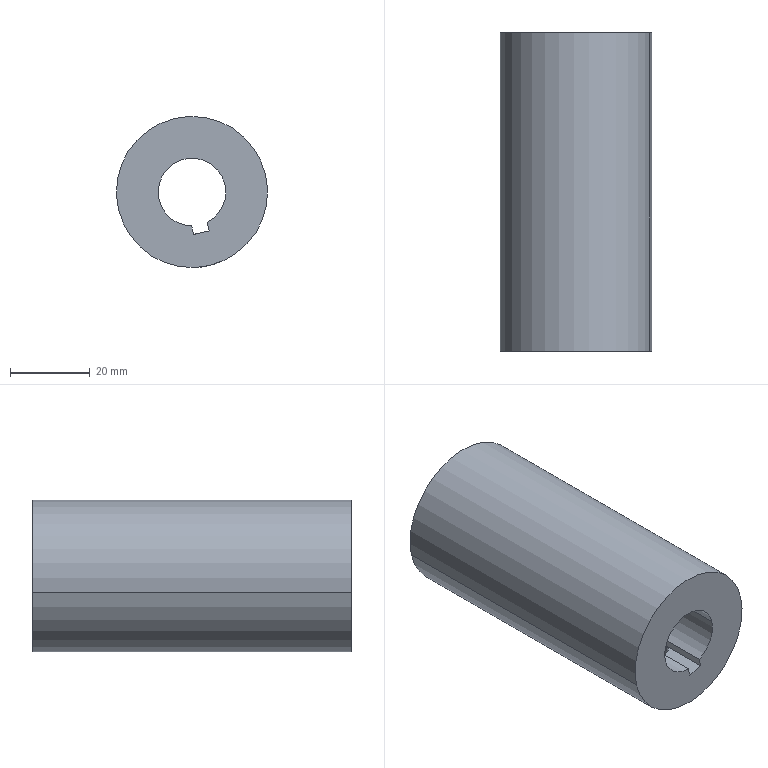Component | SolidWorks | Coupling1-1 | 1 solid | 20 faces | box 38 x 80 x 38 mm | volume 71671 mm3 | plane 11 | cylinder 9 | commonest cylinder face diameters 4.2 x4 17 x3 38 x2
build123d program:
from build123d import *

# Parameters (mm, degrees)
SKETCH1_R                  = 19
EXTRUDE1_DEPTH             = 80
M5_TAPPED_HOLE1_AT_2_COUNT = 2
M5_TAPPED_HOLE1_AT_2_PITCH = 55


with BuildPart() as part:
    # Sketch1 → Extrude1 (new body)
    with BuildSketch(Plane(origin=(0, 0, 0), x_dir=(1, 0, 0), z_dir=(0, 1, 0))):
        with Locations(Location((0, 0, 0), (0, 0, 270))):
            Circle(SKETCH1_R)
        with BuildLine():
            Line((8.261, 2), (10.5, 2))
            Line((10.5, 2), (10.5, -2))
            Line((10.5, -2), (8.261, -2))
            ThreePointArc((8.261, -2), (-8.5, 0), (8.261, 2))
        make_face(mode=Mode.SUBTRACT)
    extrude(amount=EXTRUDE1_DEPTH)

    # Sketch2 → M5 Tapped Hole1 (revolve, cut)
    with BuildSketch(Plane(origin=(10.5, 67.5, 0), x_dir=(0, 0, 1), z_dir=(0, 1, 0))):
        Polygon((0, 0), (0, 15.262), (2.1, 14), (2.1, 0), align=None)
    m5_tapped_hole1 = revolve(axis=Axis((4.15, 67.5, 0), (1, 0, 0)), mode=Mode.SUBTRACT)

    # M5 Tapped Hole1 at 2: M5 Tapped Hole1 ×2
    with Locations(*[(0, -i * M5_TAPPED_HOLE1_AT_2_PITCH, 0) for i in range(1, M5_TAPPED_HOLE1_AT_2_COUNT)]):
        add(m5_tapped_hole1, mode=Mode.SUBTRACT)


solid = part.part

# Placed as in the assembly
solid = solid.moved(Location((-164.784, 235.983, 4), (0, 77.072, 0)))
STEP:
#1=CARTESIAN_POINT('',(-6.402,11.948,-0.5856));
#2=VERTEX_POINT('',#1);
#3=CARTESIAN_POINT('',(-6.241,11.948,-0.5486));
#4=VERTEX_POINT('',#3);
#5=CARTESIAN_POINT('',(-6.402,11.948,-0.5856));
#6=CARTESIAN_POINT('',(-6.402,11.937,-0.5856));
#7=CARTESIAN_POINT('',(-6.4,11.926,-0.5854));
#8=CARTESIAN_POINT('',(-6.391,11.907,-0.5843));
#9=CARTESIAN_POINT('',(-6.385,11.897,-0.5836));
#10=CARTESIAN_POINT('',(-6.374,11.886,-0.5819));
#11=CARTESIAN_POINT('',(-6.37,11.882,-0.5812));
#12=CARTESIAN_POINT('',(-6.361,11.876,-0.5797));
#13=CARTESIAN_POINT('',(-6.356,11.874,-0.5789));
#14=CARTESIAN_POINT('',(-6.346,11.87,-0.5771));
#15=CARTESIAN_POINT('',(-6.341,11.868,-0.5761));
#16=CARTESIAN_POINT('',(-6.331,11.866,-0.574));
#17=CARTESIAN_POINT('',(-6.325,11.865,-0.5728));
#18=CARTESIAN_POINT('',(-6.315,11.865,-0.5704));
#19=CARTESIAN_POINT('',(-6.31,11.866,-0.5691));
#20=CARTESIAN_POINT('',(-6.299,11.868,-0.5665));
#21=CARTESIAN_POINT('',(-6.294,11.87,-0.5652));
#22=CARTESIAN_POINT('',(-6.285,11.874,-0.5625));
#23=CARTESIAN_POINT('',(-6.28,11.876,-0.5612));
#24=CARTESIAN_POINT('',(-6.271,11.882,-0.5587));
#25=CARTESIAN_POINT('',(-6.267,11.886,-0.5574));
#26=CARTESIAN_POINT('',(-6.256,11.897,-0.554));
#27=CARTESIAN_POINT('',(-6.251,11.906,-0.552));
#28=CARTESIAN_POINT('',(-6.243,11.926,-0.5493));
#29=CARTESIAN_POINT('',(-6.241,11.937,-0.5486));
#30=CARTESIAN_POINT('',(-6.241,11.948,-0.5486));
#31=B_SPLINE_CURVE_WITH_KNOTS('',3,(#5,#6,#7,#8,#9,#10,#11,#12,#13,#14,#15,#16,#17,#18,#19,#20,#21,#22,#23,#24,#25,#26,#27,#28,#29,#30),.UNSPECIFIED.,.F.,.F.,(4,2,2,2,2,2,2,2,2,2,2,2,4),(0.006571,0.007392,0.008213,0.008623,0.009034,0.009445,0.009855,0.01027,0.01068,0.01109,0.0115,0.01232,0.01314),.UNSPECIFIED.);
#32=EDGE_CURVE('',#2,#4,#31,.T.);
#33=ORIENTED_EDGE('',*,*,#32,.F.);
#34=CARTESIAN_POINT('',(-6.476,11.948,-0.2639));
#35=VERTEX_POINT('',#34);
#36=CARTESIAN_POINT('',(-6.476,11.948,-0.2639));
#37=DIRECTION('',(-0.2238,0.,0.9746));
#38=VECTOR('',#37,39.37);
#39=LINE('',#36,#38);
#40=EDGE_CURVE('',#2,#35,#39,.T.);
#41=ORIENTED_EDGE('',*,*,#40,.T.);
#42=CARTESIAN_POINT('',(-6.472,11.923,-0.263));
#43=VERTEX_POINT('',#42);
#44=CARTESIAN_POINT('',(-6.395,11.948,-0.2454));
#45=DIRECTION('',(-0.2238,0.,0.9746));
#46=DIRECTION('',(0.9746,0.,0.2238));
#47=AXIS2_PLACEMENT_3D('',#44,#45,#46);
#48=CIRCLE('',#47,0.08268);
#49=EDGE_CURVE('',#35,#43,#48,.T.);
#50=ORIENTED_EDGE('',*,*,#49,.T.);
#51=CARTESIAN_POINT('',(-6.318,11.923,-0.2278));
#52=VERTEX_POINT('',#51);
#53=CARTESIAN_POINT('',(-6.395,11.948,-0.2454));
#54=DIRECTION('',(-0.2238,0.,0.9746));
#55=DIRECTION('',(0.9746,0.,0.2238));
#56=AXIS2_PLACEMENT_3D('',#53,#54,#55);
#57=CIRCLE('',#56,0.08268);
#58=EDGE_CURVE('',#43,#52,#57,.T.);
#59=ORIENTED_EDGE('',*,*,#58,.T.);
#60=CARTESIAN_POINT('',(-6.314,11.948,-0.2269));
#61=VERTEX_POINT('',#60);
#62=CARTESIAN_POINT('',(-6.395,11.948,-0.2454));
#63=DIRECTION('',(-0.2238,0.,0.9746));
#64=DIRECTION('',(0.9746,0.,0.2238));
#65=AXIS2_PLACEMENT_3D('',#62,#63,#64);
#66=CIRCLE('',#65,0.08268);
#67=EDGE_CURVE('',#52,#61,#66,.T.);
#68=ORIENTED_EDGE('',*,*,#67,.T.);
#69=CARTESIAN_POINT('',(-6.314,11.948,-0.2269));
#70=DIRECTION('',(-0.2238,0.,0.9746));
#71=VECTOR('',#70,39.37);
#72=LINE('',#69,#71);
#73=EDGE_CURVE('',#4,#61,#72,.T.);
#74=ORIENTED_EDGE('',*,*,#73,.F.);
#75=EDGE_LOOP('',(#33,#41,#50,#59,#68,#74));
#76=FACE_OUTER_BOUND('',#75,.T.);
#77=CARTESIAN_POINT('',(-6.395,11.948,-0.2454));
#78=DIRECTION('',(-0.2238,0.,0.9746));
#79=DIRECTION('',(0.9746,0.,0.2238));
#80=AXIS2_PLACEMENT_3D('',#77,#78,#79);
#81=CYLINDRICAL_SURFACE('',#80,0.08268);
#82=ADVANCED_FACE('',(#76),#81,.F.);
#83=CARTESIAN_POINT('',(-6.402,9.783,-0.5856));
#84=VERTEX_POINT('',#83);
#85=CARTESIAN_POINT('',(-6.241,9.783,-0.5486));
#86=VERTEX_POINT('',#85);
#87=CARTESIAN_POINT('',(-6.402,9.783,-0.5856));
#88=CARTESIAN_POINT('',(-6.402,9.772,-0.5856));
#89=CARTESIAN_POINT('',(-6.4,9.761,-0.5854));
#90=CARTESIAN_POINT('',(-6.391,9.741,-0.5843));
#91=CARTESIAN_POINT('',(-6.385,9.732,-0.5836));
#92=CARTESIAN_POINT('',(-6.374,9.721,-0.5819));
#93=CARTESIAN_POINT('',(-6.37,9.717,-0.5812));
#94=CARTESIAN_POINT('',(-6.361,9.711,-0.5797));
#95=CARTESIAN_POINT('',(-6.356,9.709,-0.5789));
#96=CARTESIAN_POINT('',(-6.346,9.704,-0.5771));
#97=CARTESIAN_POINT('',(-6.341,9.703,-0.5761));
#98=CARTESIAN_POINT('',(-6.331,9.701,-0.574));
#99=CARTESIAN_POINT('',(-6.325,9.7,-0.5728));
#100=CARTESIAN_POINT('',(-6.315,9.7,-0.5704));
#101=CARTESIAN_POINT('',(-6.31,9.701,-0.5691));
#102=CARTESIAN_POINT('',(-6.299,9.703,-0.5665));
#103=CARTESIAN_POINT('',(-6.294,9.704,-0.5652));
#104=CARTESIAN_POINT('',(-6.285,9.708,-0.5625));
#105=CARTESIAN_POINT('',(-6.28,9.711,-0.5612));
#106=CARTESIAN_POINT('',(-6.271,9.717,-0.5587));
#107=CARTESIAN_POINT('',(-6.267,9.721,-0.5574));
#108=CARTESIAN_POINT('',(-6.256,9.732,-0.554));
#109=CARTESIAN_POINT('',(-6.251,9.741,-0.552));
#110=CARTESIAN_POINT('',(-6.243,9.761,-0.5493));
#111=CARTESIAN_POINT('',(-6.241,9.772,-0.5486));
#112=CARTESIAN_POINT('',(-6.241,9.783,-0.5486));
#113=B_SPLINE_CURVE_WITH_KNOTS('',3,(#87,#88,#89,#90,#91,#92,#93,#94,#95,#96,#97,#98,#99,#100,#101,#102,#103,#104,#105,#106,#107,#108,#109,#110,#111,#112),.UNSPECIFIED.,.F.,.F.,(4,2,2,2,2,2,2,2,2,2,2,2,4),(0.006571,0.007392,0.008213,0.008623,0.009034,0.009445,0.009855,0.01027,0.01068,0.01109,0.0115,0.01232,0.01314),.UNSPECIFIED.);
#114=EDGE_CURVE('',#84,#86,#113,.T.);
#115=ORIENTED_EDGE('',*,*,#114,.F.);
#116=CARTESIAN_POINT('',(-6.476,9.783,-0.2639));
#117=VERTEX_POINT('',#116);
#118=CARTESIAN_POINT('',(-6.476,9.783,-0.2639));
#119=DIRECTION('',(-0.2238,0.,0.9746));
#120=VECTOR('',#119,39.37);
#121=LINE('',#118,#120);
#122=EDGE_CURVE('',#84,#117,#121,.T.);
#123=ORIENTED_EDGE('',*,*,#122,.T.);
#124=CARTESIAN_POINT('',(-6.472,9.758,-0.263));
#125=VERTEX_POINT('',#124);
#126=CARTESIAN_POINT('',(-6.395,9.783,-0.2454));
#127=DIRECTION('',(-0.2238,0.,0.9746));
#128=DIRECTION('',(0.9746,0.,0.2238));
#129=AXIS2_PLACEMENT_3D('',#126,#127,#128);
#130=CIRCLE('',#129,0.08268);
#131=EDGE_CURVE('',#117,#125,#130,.T.);
#132=ORIENTED_EDGE('',*,*,#131,.T.);
#133=CARTESIAN_POINT('',(-6.318,9.758,-0.2278));
#134=VERTEX_POINT('',#133);
#135=CARTESIAN_POINT('',(-6.395,9.783,-0.2454));
#136=DIRECTION('',(-0.2238,0.,0.9746));
#137=DIRECTION('',(0.9746,0.,0.2238));
#138=AXIS2_PLACEMENT_3D('',#135,#136,#137);
#139=CIRCLE('',#138,0.08268);
#140=EDGE_CURVE('',#125,#134,#139,.T.);
#141=ORIENTED_EDGE('',*,*,#140,.T.);
#142=CARTESIAN_POINT('',(-6.314,9.783,-0.2269));
#143=VERTEX_POINT('',#142);
#144=CARTESIAN_POINT('',(-6.395,9.783,-0.2454));
#145=DIRECTION('',(-0.2238,0.,0.9746));
#146=DIRECTION('',(0.9746,0.,0.2238));
#147=AXIS2_PLACEMENT_3D('',#144,#145,#146);
#148=CIRCLE('',#147,0.08268);
#149=EDGE_CURVE('',#134,#143,#148,.T.);
#150=ORIENTED_EDGE('',*,*,#149,.T.);
#151=CARTESIAN_POINT('',(-6.314,9.783,-0.2269));
#152=DIRECTION('',(-0.2238,0.,0.9746));
#153=VECTOR('',#152,39.37);
#154=LINE('',#151,#153);
#155=EDGE_CURVE('',#86,#143,#154,.T.);
#156=ORIENTED_EDGE('',*,*,#155,.F.);
#157=EDGE_LOOP('',(#115,#123,#132,#141,#150,#156));
#158=FACE_OUTER_BOUND('',#157,.T.);
#159=CARTESIAN_POINT('',(-6.395,9.783,-0.2454));
#160=DIRECTION('',(-0.2238,0.,0.9746));
#161=DIRECTION('',(0.9746,0.,0.2238));
#162=AXIS2_PLACEMENT_3D('',#159,#160,#161);
#163=CYLINDRICAL_SURFACE('',#162,0.08268);
#164=ADVANCED_FACE('',(#158),#163,.F.);
#165=CARTESIAN_POINT('',(-6.814,12.44,0.08257));
#166=VERTEX_POINT('',#165);
#167=CARTESIAN_POINT('',(-6.161,12.44,0.2324));
#168=VERTEX_POINT('',#167);
#169=CARTESIAN_POINT('',(-6.488,12.44,0.1575));
#170=DIRECTION('',(0.,1.,0.));
#171=DIRECTION('',(0.9746,0.,0.2238));
#172=AXIS2_PLACEMENT_3D('',#169,#170,#171);
#173=CIRCLE('',#172,0.3346);
#174=EDGE_CURVE('',#166,#168,#173,.T.);
#175=ORIENTED_EDGE('',*,*,#174,.T.);
#176=CARTESIAN_POINT('',(-6.161,9.291,0.2324));
#177=VERTEX_POINT('',#176);
#178=CARTESIAN_POINT('',(-6.161,12.44,0.2324));
#179=DIRECTION('',(0.,-1.,0.));
#180=VECTOR('',#179,39.37);
#181=LINE('',#178,#180);
#182=EDGE_CURVE('',#168,#177,#181,.T.);
#183=ORIENTED_EDGE('',*,*,#182,.T.);
#184=CARTESIAN_POINT('',(-6.814,9.291,0.08257));
#185=VERTEX_POINT('',#184);
#186=CARTESIAN_POINT('',(-6.488,9.291,0.1575));
#187=DIRECTION('',(0.,1.,0.));
#188=DIRECTION('',(0.9746,0.,0.2238));
#189=AXIS2_PLACEMENT_3D('',#186,#187,#188);
#190=CIRCLE('',#189,0.3346);
#191=EDGE_CURVE('',#185,#177,#190,.T.);
#192=ORIENTED_EDGE('',*,*,#191,.F.);
#193=CARTESIAN_POINT('',(-6.814,12.44,0.08257));
#194=DIRECTION('',(0.,-1.,0.));
#195=VECTOR('',#194,39.37);
#196=LINE('',#193,#195);
#197=EDGE_CURVE('',#166,#185,#196,.T.);
#198=ORIENTED_EDGE('',*,*,#197,.F.);
#199=EDGE_LOOP('',(#175,#183,#192,#198));
#200=FACE_OUTER_BOUND('',#199,.T.);
#201=CARTESIAN_POINT('',(-6.488,12.44,0.1575));
#202=DIRECTION('',(0.,-1.,0.));
#203=DIRECTION('',(-0.9746,0.,-0.2238));
#204=AXIS2_PLACEMENT_3D('',#201,#202,#203);
#205=CYLINDRICAL_SURFACE('',#204,0.3346);
#206=ADVANCED_FACE('',(#200),#205,.F.);
#207=CARTESIAN_POINT('',(-6.491,12.44,-0.1771));
#208=VERTEX_POINT('',#207);
#209=CARTESIAN_POINT('',(-6.488,12.44,0.1575));
#210=DIRECTION('',(0.,1.,0.));
#211=DIRECTION('',(0.9746,0.,0.2238));
#212=AXIS2_PLACEMENT_3D('',#209,#210,#211);
#213=CIRCLE('',#212,0.3346);
#214=EDGE_CURVE('',#208,#166,#213,.T.);
#215=ORIENTED_EDGE('',*,*,#214,.T.);
#216=ORIENTED_EDGE('',*,*,#197,.T.);
#217=CARTESIAN_POINT('',(-6.491,9.291,-0.1771));
#218=VERTEX_POINT('',#217);
#219=CARTESIAN_POINT('',(-6.488,9.291,0.1575));
#220=DIRECTION('',(0.,1.,0.));
#221=DIRECTION('',(0.9746,0.,0.2238));
#222=AXIS2_PLACEMENT_3D('',#219,#220,#221);
#223=CIRCLE('',#222,0.3346);
#224=EDGE_CURVE('',#218,#185,#223,.T.);
#225=ORIENTED_EDGE('',*,*,#224,.F.);
#226=CARTESIAN_POINT('',(-6.491,12.44,-0.1771));
#227=DIRECTION('',(0.,-1.,0.));
#228=VECTOR('',#227,39.37);
#229=LINE('',#226,#228);
#230=EDGE_CURVE('',#208,#218,#229,.T.);
#231=ORIENTED_EDGE('',*,*,#230,.F.);
#232=EDGE_LOOP('',(#215,#216,#225,#231));
#233=FACE_OUTER_BOUND('',#232,.T.);
#234=CARTESIAN_POINT('',(-6.488,12.44,0.1575));
#235=DIRECTION('',(0.,-1.,0.));
#236=DIRECTION('',(-0.9746,0.,-0.2238));
#237=AXIS2_PLACEMENT_3D('',#234,#235,#236);
#238=CYLINDRICAL_SURFACE('',#237,0.3346);
#239=ADVANCED_FACE('',(#233),#238,.F.);
#240=CARTESIAN_POINT('',(-6.241,11.948,-0.5486));
#241=CARTESIAN_POINT('',(-6.241,11.954,-0.5486));
#242=CARTESIAN_POINT('',(-6.241,11.959,-0.5488));
#243=CARTESIAN_POINT('',(-6.243,11.97,-0.5495));
#244=CARTESIAN_POINT('',(-6.245,11.975,-0.55));
#245=CARTESIAN_POINT('',(-6.249,11.985,-0.5513));
#246=CARTESIAN_POINT('',(-6.251,11.99,-0.5522));
#247=CARTESIAN_POINT('',(-6.257,11.999,-0.554));
#248=CARTESIAN_POINT('',(-6.26,12.003,-0.5551));
#249=CARTESIAN_POINT('',(-6.271,12.014,-0.5585));
#250=CARTESIAN_POINT('',(-6.28,12.02,-0.5612));
#251=CARTESIAN_POINT('',(-6.299,12.029,-0.5665));
#252=CARTESIAN_POINT('',(-6.31,12.031,-0.5691));
#253=CARTESIAN_POINT('',(-6.325,12.031,-0.5728));
#254=CARTESIAN_POINT('',(-6.331,12.03,-0.5739));
#255=CARTESIAN_POINT('',(-6.341,12.028,-0.5761));
#256=CARTESIAN_POINT('',(-6.346,12.027,-0.5771));
#257=CARTESIAN_POINT('',(-6.356,12.022,-0.5789));
#258=CARTESIAN_POINT('',(-6.361,12.02,-0.5797));
#259=CARTESIAN_POINT('',(-6.37,12.014,-0.5812));
#260=CARTESIAN_POINT('',(-6.374,12.01,-0.5819));
#261=CARTESIAN_POINT('',(-6.381,12.003,-0.583));
#262=CARTESIAN_POINT('',(-6.385,11.999,-0.5835));
#263=CARTESIAN_POINT('',(-6.391,11.99,-0.5843));
#264=CARTESIAN_POINT('',(-6.393,11.985,-0.5846));
#265=CARTESIAN_POINT('',(-6.397,11.975,-0.5851));
#266=CARTESIAN_POINT('',(-6.399,11.97,-0.5853));
#267=CARTESIAN_POINT('',(-6.401,11.959,-0.5855));
#268=CARTESIAN_POINT('',(-6.402,11.954,-0.5856));
#269=CARTESIAN_POINT('',(-6.402,11.948,-0.5856));
#270=B_SPLINE_CURVE_WITH_KNOTS('',3,(#240,#241,#242,#243,#244,#245,#246,#247,#248,#249,#250,#251,#252,#253,#254,#255,#256,#257,#258,#259,#260,#261,#262,#263,#264,#265,#266,#267,#268,#269),.UNSPECIFIED.,.F.,.F.,(4,2,2,2,2,2,2,2,2,2,2,2,2,2,4),(0.,0.0004107,0.0008213,0.001232,0.001643,0.002464,0.003285,0.003696,0.004107,0.004517,0.004928,0.005339,0.005749,0.00616,0.006571),.UNSPECIFIED.);
#271=EDGE_CURVE('',#4,#2,#270,.T.);
#272=ORIENTED_EDGE('',*,*,#271,.T.);
#273=ORIENTED_EDGE('',*,*,#32,.T.);
#274=EDGE_LOOP('',(#272,#273));
#275=FACE_BOUND('',#274,.T.);
#276=CARTESIAN_POINT('',(-6.241,9.783,-0.5486));
#277=CARTESIAN_POINT('',(-6.241,9.788,-0.5486));
#278=CARTESIAN_POINT('',(-6.241,9.794,-0.5488));
#279=CARTESIAN_POINT('',(-6.243,9.804,-0.5495));
#280=CARTESIAN_POINT('',(-6.245,9.809,-0.55));
#281=CARTESIAN_POINT('',(-6.249,9.819,-0.5513));
#282=CARTESIAN_POINT('',(-6.251,9.824,-0.5522));
#283=CARTESIAN_POINT('',(-6.257,9.833,-0.554));
#284=CARTESIAN_POINT('',(-6.26,9.837,-0.5551));
#285=CARTESIAN_POINT('',(-6.271,9.849,-0.5585));
#286=CARTESIAN_POINT('',(-6.28,9.855,-0.5612));
#287=CARTESIAN_POINT('',(-6.299,9.863,-0.5665));
#288=CARTESIAN_POINT('',(-6.31,9.865,-0.5691));
#289=CARTESIAN_POINT('',(-6.325,9.865,-0.5728));
#290=CARTESIAN_POINT('',(-6.331,9.865,-0.5739));
#291=CARTESIAN_POINT('',(-6.341,9.863,-0.5761));
#292=CARTESIAN_POINT('',(-6.346,9.861,-0.5771));
#293=CARTESIAN_POINT('',(-6.356,9.857,-0.5789));
#294=CARTESIAN_POINT('',(-6.361,9.855,-0.5797));
#295=CARTESIAN_POINT('',(-6.37,9.849,-0.5812));
#296=CARTESIAN_POINT('',(-6.374,9.845,-0.5819));
#297=CARTESIAN_POINT('',(-6.381,9.837,-0.583));
#298=CARTESIAN_POINT('',(-6.385,9.833,-0.5835));
#299=CARTESIAN_POINT('',(-6.391,9.824,-0.5843));
#300=CARTESIAN_POINT('',(-6.393,9.819,-0.5846));
#301=CARTESIAN_POINT('',(-6.397,9.809,-0.5851));
#302=CARTESIAN_POINT('',(-6.399,9.804,-0.5853));
#303=CARTESIAN_POINT('',(-6.401,9.794,-0.5855));
#304=CARTESIAN_POINT('',(-6.402,9.788,-0.5856));
#305=CARTESIAN_POINT('',(-6.402,9.783,-0.5856));
#306=B_SPLINE_CURVE_WITH_KNOTS('',3,(#276,#277,#278,#279,#280,#281,#282,#283,#284,#285,#286,#287,#288,#289,#290,#291,#292,#293,#294,#295,#296,#297,#298,#299,#300,#301,#302,#303,#304,#305),.UNSPECIFIED.,.F.,.F.,(4,2,2,2,2,2,2,2,2,2,2,2,2,2,4),(0.,0.0004107,0.0008213,0.001232,0.001643,0.002464,0.003285,0.003696,0.004107,0.004517,0.004928,0.005339,0.005749,0.00616,0.006571),.UNSPECIFIED.);
#307=EDGE_CURVE('',#86,#84,#306,.T.);
#308=ORIENTED_EDGE('',*,*,#307,.T.);
#309=ORIENTED_EDGE('',*,*,#114,.T.);
#310=EDGE_LOOP('',(#308,#309));
#311=FACE_BOUND('',#310,.T.);
#312=CARTESIAN_POINT('',(-5.758,12.44,0.3249));
#313=VERTEX_POINT('',#312);
#314=CARTESIAN_POINT('',(-7.217,12.44,-0.009957));
#315=VERTEX_POINT('',#314);
#316=CARTESIAN_POINT('',(-6.488,12.44,0.1575));
#317=DIRECTION('',(0.,1.,0.));
#318=DIRECTION('',(0.9746,0.,0.2238));
#319=AXIS2_PLACEMENT_3D('',#316,#317,#318);
#320=CIRCLE('',#319,0.748);
#321=EDGE_CURVE('',#313,#315,#320,.T.);
#322=ORIENTED_EDGE('',*,*,#321,.F.);
#323=CARTESIAN_POINT('',(-5.758,9.291,0.3249));
#324=VERTEX_POINT('',#323);
#325=CARTESIAN_POINT('',(-5.758,12.44,0.3249));
#326=DIRECTION('',(0.,-1.,0.));
#327=VECTOR('',#326,39.37);
#328=LINE('',#325,#327);
#329=EDGE_CURVE('',#313,#324,#328,.T.);
#330=ORIENTED_EDGE('',*,*,#329,.T.);
#331=CARTESIAN_POINT('',(-7.217,9.291,-0.009957));
#332=VERTEX_POINT('',#331);
#333=CARTESIAN_POINT('',(-6.488,9.291,0.1575));
#334=DIRECTION('',(0.,1.,0.));
#335=DIRECTION('',(0.9746,0.,0.2238));
#336=AXIS2_PLACEMENT_3D('',#333,#334,#335);
#337=CIRCLE('',#336,0.748);
#338=EDGE_CURVE('',#324,#332,#337,.T.);
#339=ORIENTED_EDGE('',*,*,#338,.T.);
#340=CARTESIAN_POINT('',(-7.217,12.44,-0.009957));
#341=DIRECTION('',(0.,-1.,0.));
#342=VECTOR('',#341,39.37);
#343=LINE('',#340,#342);
#344=EDGE_CURVE('',#315,#332,#343,.T.);
#345=ORIENTED_EDGE('',*,*,#344,.F.);
#346=EDGE_LOOP('',(#322,#330,#339,#345));
#347=FACE_OUTER_BOUND('',#346,.T.);
#348=CARTESIAN_POINT('',(-6.488,12.44,0.1575));
#349=DIRECTION('',(0.,-1.,0.));
#350=DIRECTION('',(-0.9746,0.,-0.2238));
#351=AXIS2_PLACEMENT_3D('',#348,#349,#350);
#352=CYLINDRICAL_SURFACE('',#351,0.748);
#353=ADVANCED_FACE('',(#275,#311,#347),#352,.T.);
#354=CARTESIAN_POINT('',(-6.318,11.973,-0.2278));
#355=VERTEX_POINT('',#354);
#356=CARTESIAN_POINT('',(-6.472,11.973,-0.263));
#357=VERTEX_POINT('',#356);
#358=CARTESIAN_POINT('',(-6.395,11.948,-0.2454));
#359=DIRECTION('',(-0.2238,0.,0.9746));
#360=DIRECTION('',(0.9746,0.,0.2238));
#361=AXIS2_PLACEMENT_3D('',#358,#359,#360);
#362=CIRCLE('',#361,0.08268);
#363=EDGE_CURVE('',#355,#357,#362,.T.);
#364=ORIENTED_EDGE('',*,*,#363,.F.);
#365=CARTESIAN_POINT('',(-6.318,12.44,-0.2278));
#366=VERTEX_POINT('',#365);
#367=CARTESIAN_POINT('',(-6.318,12.44,-0.2278));
#368=DIRECTION('',(0.,-1.,0.));
#369=VECTOR('',#368,39.37);
#370=LINE('',#367,#369);
#371=EDGE_CURVE('',#366,#355,#370,.T.);
#372=ORIENTED_EDGE('',*,*,#371,.F.);
#373=CARTESIAN_POINT('',(-6.472,12.44,-0.263));
#374=VERTEX_POINT('',#373);
#375=CARTESIAN_POINT('',(-6.472,12.44,-0.263));
#376=DIRECTION('',(-0.9746,0.,-0.2238));
#377=VECTOR('',#376,39.37);
#378=LINE('',#375,#377);
#379=EDGE_CURVE('',#366,#374,#378,.T.);
#380=ORIENTED_EDGE('',*,*,#379,.T.);
#381=CARTESIAN_POINT('',(-6.472,12.44,-0.263));
#382=DIRECTION('',(0.,-1.,0.));
#383=VECTOR('',#382,39.37);
#384=LINE('',#381,#383);
#385=EDGE_CURVE('',#374,#357,#384,.T.);
#386=ORIENTED_EDGE('',*,*,#385,.T.);
#387=EDGE_LOOP('',(#364,#372,#380,#386));
#388=FACE_OUTER_BOUND('',#387,.T.);
#389=CARTESIAN_POINT('',(-6.472,12.44,-0.263));
#390=DIRECTION('',(-0.2238,0.,0.9746));
#391=DIRECTION('',(0.9746,0.,0.2238));
#392=AXIS2_PLACEMENT_3D('',#389,#390,#391);
#393=PLANE('',#392);
#394=ADVANCED_FACE('',(#388),#393,.T.);
#395=ORIENTED_EDGE('',*,*,#58,.F.);
#396=CARTESIAN_POINT('',(-6.472,9.808,-0.263));
#397=VERTEX_POINT('',#396);
#398=CARTESIAN_POINT('',(-6.472,12.44,-0.263));
#399=DIRECTION('',(0.,-1.,0.));
#400=VECTOR('',#399,39.37);
#401=LINE('',#398,#400);
#402=EDGE_CURVE('',#43,#397,#401,.T.);
#403=ORIENTED_EDGE('',*,*,#402,.T.);
#404=CARTESIAN_POINT('',(-6.318,9.808,-0.2278));
#405=VERTEX_POINT('',#404);
#406=CARTESIAN_POINT('',(-6.395,9.783,-0.2454));
#407=DIRECTION('',(-0.2238,0.,0.9746));
#408=DIRECTION('',(0.9746,0.,0.2238));
#409=AXIS2_PLACEMENT_3D('',#406,#407,#408);
#410=CIRCLE('',#409,0.08268);
#411=EDGE_CURVE('',#405,#397,#410,.T.);
#412=ORIENTED_EDGE('',*,*,#411,.F.);
#413=CARTESIAN_POINT('',(-6.318,12.44,-0.2278));
#414=DIRECTION('',(0.,-1.,0.));
#415=VECTOR('',#414,39.37);
#416=LINE('',#413,#415);
#417=EDGE_CURVE('',#52,#405,#416,.T.);
#418=ORIENTED_EDGE('',*,*,#417,.F.);
#419=EDGE_LOOP('',(#395,#403,#412,#418));
#420=FACE_OUTER_BOUND('',#419,.T.);
#421=CARTESIAN_POINT('',(-6.472,12.44,-0.263));
#422=DIRECTION('',(-0.2238,0.,0.9746));
#423=DIRECTION('',(0.9746,0.,0.2238));
#424=AXIS2_PLACEMENT_3D('',#421,#422,#423);
#425=PLANE('',#424);
#426=ADVANCED_FACE('',(#420),#425,.T.);
#427=CARTESIAN_POINT('',(-6.488,12.44,0.1575));
#428=DIRECTION('',(0.,1.,0.));
#429=DIRECTION('',(0.9746,0.,0.2238));
#430=AXIS2_PLACEMENT_3D('',#427,#428,#429);
#431=CIRCLE('',#430,0.748);
#432=EDGE_CURVE('',#315,#313,#431,.T.);
#433=ORIENTED_EDGE('',*,*,#432,.T.);
#434=ORIENTED_EDGE('',*,*,#321,.T.);
#435=EDGE_LOOP('',(#433,#434));
#436=FACE_OUTER_BOUND('',#435,.T.);
#437=CARTESIAN_POINT('',(-6.491,12.44,-0.1771));
#438=DIRECTION('',(-0.2238,0.,0.9746));
#439=VECTOR('',#438,39.37);
#440=LINE('',#437,#439);
#441=EDGE_CURVE('',#374,#208,#440,.T.);
#442=ORIENTED_EDGE('',*,*,#441,.F.);
#443=ORIENTED_EDGE('',*,*,#379,.F.);
#444=CARTESIAN_POINT('',(-6.338,12.44,-0.1419));
#445=VERTEX_POINT('',#444);
#446=CARTESIAN_POINT('',(-6.338,12.44,-0.1419));
#447=DIRECTION('',(0.2238,0.,-0.9746));
#448=VECTOR('',#447,39.37);
#449=LINE('',#446,#448);
#450=EDGE_CURVE('',#445,#366,#449,.T.);
#451=ORIENTED_EDGE('',*,*,#450,.F.);
#452=CARTESIAN_POINT('',(-6.488,12.44,0.1575));
#453=DIRECTION('',(0.,1.,0.));
#454=DIRECTION('',(0.9746,0.,0.2238));
#455=AXIS2_PLACEMENT_3D('',#452,#453,#454);
#456=CIRCLE('',#455,0.3346);
#457=EDGE_CURVE('',#168,#445,#456,.T.);
#458=ORIENTED_EDGE('',*,*,#457,.F.);
#459=ORIENTED_EDGE('',*,*,#174,.F.);
#460=ORIENTED_EDGE('',*,*,#214,.F.);
#461=EDGE_LOOP('',(#442,#443,#451,#458,#459,#460));
#462=FACE_BOUND('',#461,.T.);
#463=CARTESIAN_POINT('',(-6.488,12.44,0.1575));
#464=DIRECTION('',(0.,1.,0.));
#465=DIRECTION('',(0.9746,0.,0.2238));
#466=AXIS2_PLACEMENT_3D('',#463,#464,#465);
#467=PLANE('',#466);
#468=ADVANCED_FACE('',(#436,#462),#467,.T.);
#469=CARTESIAN_POINT('',(-6.488,9.291,0.1575));
#470=DIRECTION('',(0.,1.,0.));
#471=DIRECTION('',(0.9746,0.,0.2238));
#472=AXIS2_PLACEMENT_3D('',#469,#470,#471);
#473=CIRCLE('',#472,0.748);
#474=EDGE_CURVE('',#332,#324,#473,.T.);
#475=ORIENTED_EDGE('',*,*,#474,.F.);
#476=ORIENTED_EDGE('',*,*,#338,.F.);
#477=EDGE_LOOP('',(#475,#476));
#478=FACE_OUTER_BOUND('',#477,.T.);
#479=CARTESIAN_POINT('',(-6.318,9.291,-0.2278));
#480=VERTEX_POINT('',#479);
#481=CARTESIAN_POINT('',(-6.472,9.291,-0.263));
#482=VERTEX_POINT('',#481);
#483=CARTESIAN_POINT('',(-6.472,9.291,-0.263));
#484=DIRECTION('',(-0.9746,0.,-0.2238));
#485=VECTOR('',#484,39.37);
#486=LINE('',#483,#485);
#487=EDGE_CURVE('',#480,#482,#486,.T.);
#488=ORIENTED_EDGE('',*,*,#487,.T.);
#489=CARTESIAN_POINT('',(-6.491,9.291,-0.1771));
#490=DIRECTION('',(-0.2238,0.,0.9746));
#491=VECTOR('',#490,39.37);
#492=LINE('',#489,#491);
#493=EDGE_CURVE('',#482,#218,#492,.T.);
#494=ORIENTED_EDGE('',*,*,#493,.T.);
#495=ORIENTED_EDGE('',*,*,#224,.T.);
#496=ORIENTED_EDGE('',*,*,#191,.T.);
#497=CARTESIAN_POINT('',(-6.338,9.291,-0.1419));
#498=VERTEX_POINT('',#497);
#499=CARTESIAN_POINT('',(-6.488,9.291,0.1575));
#500=DIRECTION('',(0.,1.,0.));
#501=DIRECTION('',(0.9746,0.,0.2238));
#502=AXIS2_PLACEMENT_3D('',#499,#500,#501);
#503=CIRCLE('',#502,0.3346);
#504=EDGE_CURVE('',#177,#498,#503,.T.);
#505=ORIENTED_EDGE('',*,*,#504,.T.);
#506=CARTESIAN_POINT('',(-6.338,9.291,-0.1419));
#507=DIRECTION('',(0.2238,0.,-0.9746));
#508=VECTOR('',#507,39.37);
#509=LINE('',#506,#508);
#510=EDGE_CURVE('',#498,#480,#509,.T.);
#511=ORIENTED_EDGE('',*,*,#510,.T.);
#512=EDGE_LOOP('',(#488,#494,#495,#496,#505,#511));
#513=FACE_BOUND('',#512,.T.);
#514=CARTESIAN_POINT('',(-6.488,9.291,0.1575));
#515=DIRECTION('',(0.,1.,0.));
#516=DIRECTION('',(0.9746,0.,0.2238));
#517=AXIS2_PLACEMENT_3D('',#514,#515,#516);
#518=PLANE('',#517);
#519=ADVANCED_FACE('',(#478,#513),#518,.F.);
#520=ORIENTED_EDGE('',*,*,#329,.F.);
#521=ORIENTED_EDGE('',*,*,#432,.F.);
#522=ORIENTED_EDGE('',*,*,#344,.T.);
#523=ORIENTED_EDGE('',*,*,#474,.T.);
#524=EDGE_LOOP('',(#520,#521,#522,#523));
#525=FACE_OUTER_BOUND('',#524,.T.);
#526=CARTESIAN_POINT('',(-6.488,12.44,0.1575));
#527=DIRECTION('',(0.,-1.,0.));
#528=DIRECTION('',(-0.9746,0.,-0.2238));
#529=AXIS2_PLACEMENT_3D('',#526,#527,#528);
#530=CYLINDRICAL_SURFACE('',#529,0.748);
#531=ADVANCED_FACE('',(#525),#530,.T.);
#532=ORIENTED_EDGE('',*,*,#140,.F.);
#533=CARTESIAN_POINT('',(-6.472,12.44,-0.263));
#534=DIRECTION('',(0.,-1.,0.));
#535=VECTOR('',#534,39.37);
#536=LINE('',#533,#535);
#537=EDGE_CURVE('',#125,#482,#536,.T.);
#538=ORIENTED_EDGE('',*,*,#537,.T.);
#539=ORIENTED_EDGE('',*,*,#487,.F.);
#540=CARTESIAN_POINT('',(-6.318,12.44,-0.2278));
#541=DIRECTION('',(0.,-1.,0.));
#542=VECTOR('',#541,39.37);
#543=LINE('',#540,#542);
#544=EDGE_CURVE('',#134,#480,#543,.T.);
#545=ORIENTED_EDGE('',*,*,#544,.F.);
#546=EDGE_LOOP('',(#532,#538,#539,#545));
#547=FACE_OUTER_BOUND('',#546,.T.);
#548=CARTESIAN_POINT('',(-6.472,12.44,-0.263));
#549=DIRECTION('',(-0.2238,0.,0.9746));
#550=DIRECTION('',(0.9746,0.,0.2238));
#551=AXIS2_PLACEMENT_3D('',#548,#549,#550);
#552=PLANE('',#551);
#553=ADVANCED_FACE('',(#547),#552,.T.);
#554=ORIENTED_EDGE('',*,*,#493,.F.);
#555=ORIENTED_EDGE('',*,*,#537,.F.);
#556=CARTESIAN_POINT('',(-6.472,12.44,-0.263));
#557=DIRECTION('',(0.,-1.,0.));
#558=VECTOR('',#557,39.37);
#559=LINE('',#556,#558);
#560=EDGE_CURVE('',#397,#125,#559,.T.);
#561=ORIENTED_EDGE('',*,*,#560,.F.);
#562=ORIENTED_EDGE('',*,*,#402,.F.);
#563=CARTESIAN_POINT('',(-6.472,12.44,-0.263));
#564=DIRECTION('',(0.,-1.,0.));
#565=VECTOR('',#564,39.37);
#566=LINE('',#563,#565);
#567=EDGE_CURVE('',#357,#43,#566,.T.);
#568=ORIENTED_EDGE('',*,*,#567,.F.);
#569=ORIENTED_EDGE('',*,*,#385,.F.);
#570=ORIENTED_EDGE('',*,*,#441,.T.);
#571=ORIENTED_EDGE('',*,*,#230,.T.);
#572=EDGE_LOOP('',(#554,#555,#561,#562,#568,#569,#570,#571));
#573=FACE_OUTER_BOUND('',#572,.T.);
#574=CARTESIAN_POINT('',(-6.491,12.44,-0.1771));
#575=DIRECTION('',(0.9746,0.,0.2238));
#576=DIRECTION('',(0.2238,0.,-0.9746));
#577=AXIS2_PLACEMENT_3D('',#574,#575,#576);
#578=PLANE('',#577);
#579=ADVANCED_FACE('',(#573),#578,.T.);
#580=ORIENTED_EDGE('',*,*,#182,.F.);
#581=ORIENTED_EDGE('',*,*,#457,.T.);
#582=CARTESIAN_POINT('',(-6.338,12.44,-0.1419));
#583=DIRECTION('',(0.,-1.,0.));
#584=VECTOR('',#583,39.37);
#585=LINE('',#582,#584);
#586=EDGE_CURVE('',#445,#498,#585,.T.);
#587=ORIENTED_EDGE('',*,*,#586,.T.);
#588=ORIENTED_EDGE('',*,*,#504,.F.);
#589=EDGE_LOOP('',(#580,#581,#587,#588));
#590=FACE_OUTER_BOUND('',#589,.T.);
#591=CARTESIAN_POINT('',(-6.488,12.44,0.1575));
#592=DIRECTION('',(0.,-1.,0.));
#593=DIRECTION('',(-0.9746,0.,-0.2238));
#594=AXIS2_PLACEMENT_3D('',#591,#592,#593);
#595=CYLINDRICAL_SURFACE('',#594,0.3346);
#596=ADVANCED_FACE('',(#590),#595,.F.);
#597=ORIENTED_EDGE('',*,*,#510,.F.);
#598=ORIENTED_EDGE('',*,*,#586,.F.);
#599=ORIENTED_EDGE('',*,*,#450,.T.);
#600=ORIENTED_EDGE('',*,*,#371,.T.);
#601=CARTESIAN_POINT('',(-6.318,12.44,-0.2278));
#602=DIRECTION('',(0.,-1.,0.));
#603=VECTOR('',#602,39.37);
#604=LINE('',#601,#603);
#605=EDGE_CURVE('',#355,#52,#604,.T.);
#606=ORIENTED_EDGE('',*,*,#605,.T.);
#607=ORIENTED_EDGE('',*,*,#417,.T.);
#608=CARTESIAN_POINT('',(-6.318,12.44,-0.2278));
#609=DIRECTION('',(0.,-1.,0.));
#610=VECTOR('',#609,39.37);
#611=LINE('',#608,#610);
#612=EDGE_CURVE('',#405,#134,#611,.T.);
#613=ORIENTED_EDGE('',*,*,#612,.T.);
#614=ORIENTED_EDGE('',*,*,#544,.T.);
#615=EDGE_LOOP('',(#597,#598,#599,#600,#606,#607,#613,#614));
#616=FACE_OUTER_BOUND('',#615,.T.);
#617=CARTESIAN_POINT('',(-6.338,12.44,-0.1419));
#618=DIRECTION('',(-0.9746,0.,-0.2238));
#619=DIRECTION('',(-0.2238,0.,0.9746));
#620=AXIS2_PLACEMENT_3D('',#617,#618,#619);
#621=PLANE('',#620);
#622=ADVANCED_FACE('',(#616),#621,.T.);
#623=ORIENTED_EDGE('',*,*,#560,.T.);
#624=ORIENTED_EDGE('',*,*,#131,.F.);
#625=CARTESIAN_POINT('',(-6.395,9.783,-0.2454));
#626=DIRECTION('',(-0.2238,0.,0.9746));
#627=DIRECTION('',(0.9746,0.,0.2238));
#628=AXIS2_PLACEMENT_3D('',#625,#626,#627);
#629=CIRCLE('',#628,0.08268);
#630=EDGE_CURVE('',#397,#117,#629,.T.);
#631=ORIENTED_EDGE('',*,*,#630,.F.);
#632=EDGE_LOOP('',(#623,#624,#631));
#633=FACE_OUTER_BOUND('',#632,.T.);
#634=CARTESIAN_POINT('',(-6.395,9.865,-0.2454));
#635=DIRECTION('',(-0.2238,0.,0.9746));
#636=DIRECTION('',(0.9746,0.,0.2238));
#637=AXIS2_PLACEMENT_3D('',#634,#635,#636);
#638=PLANE('',#637);
#639=ADVANCED_FACE('',(#633),#638,.F.);
#640=ORIENTED_EDGE('',*,*,#122,.F.);
#641=ORIENTED_EDGE('',*,*,#307,.F.);
#642=ORIENTED_EDGE('',*,*,#155,.T.);
#643=CARTESIAN_POINT('',(-6.395,9.783,-0.2454));
#644=DIRECTION('',(-0.2238,0.,0.9746));
#645=DIRECTION('',(0.9746,0.,0.2238));
#646=AXIS2_PLACEMENT_3D('',#643,#644,#645);
#647=CIRCLE('',#646,0.08268);
#648=EDGE_CURVE('',#143,#405,#647,.T.);
#649=ORIENTED_EDGE('',*,*,#648,.T.);
#650=ORIENTED_EDGE('',*,*,#411,.T.);
#651=ORIENTED_EDGE('',*,*,#630,.T.);
#652=EDGE_LOOP('',(#640,#641,#642,#649,#650,#651));
#653=FACE_OUTER_BOUND('',#652,.T.);
#654=CARTESIAN_POINT('',(-6.395,9.783,-0.2454));
#655=DIRECTION('',(-0.2238,0.,0.9746));
#656=DIRECTION('',(0.9746,0.,0.2238));
#657=AXIS2_PLACEMENT_3D('',#654,#655,#656);
#658=CYLINDRICAL_SURFACE('',#657,0.08268);
#659=ADVANCED_FACE('',(#653),#658,.F.);
#660=ORIENTED_EDGE('',*,*,#612,.F.);
#661=ORIENTED_EDGE('',*,*,#648,.F.);
#662=ORIENTED_EDGE('',*,*,#149,.F.);
#663=EDGE_LOOP('',(#660,#661,#662));
#664=FACE_OUTER_BOUND('',#663,.T.);
#665=CARTESIAN_POINT('',(-6.395,9.865,-0.2454));
#666=DIRECTION('',(-0.2238,0.,0.9746));
#667=DIRECTION('',(0.9746,0.,0.2238));
#668=AXIS2_PLACEMENT_3D('',#665,#666,#667);
#669=PLANE('',#668);
#670=ADVANCED_FACE('',(#664),#669,.F.);
#671=ORIENTED_EDGE('',*,*,#67,.F.);
#672=ORIENTED_EDGE('',*,*,#605,.F.);
#673=CARTESIAN_POINT('',(-6.395,11.948,-0.2454));
#674=DIRECTION('',(-0.2238,0.,0.9746));
#675=DIRECTION('',(0.9746,0.,0.2238));
#676=AXIS2_PLACEMENT_3D('',#673,#674,#675);
#677=CIRCLE('',#676,0.08268);
#678=EDGE_CURVE('',#61,#355,#677,.T.);
#679=ORIENTED_EDGE('',*,*,#678,.F.);
#680=EDGE_LOOP('',(#671,#672,#679));
#681=FACE_OUTER_BOUND('',#680,.T.);
#682=CARTESIAN_POINT('',(-6.395,12.031,-0.2454));
#683=DIRECTION('',(-0.2238,0.,0.9746));
#684=DIRECTION('',(0.9746,0.,0.2238));
#685=AXIS2_PLACEMENT_3D('',#682,#683,#684);
#686=PLANE('',#685);
#687=ADVANCED_FACE('',(#681),#686,.F.);
#688=ORIENTED_EDGE('',*,*,#40,.F.);
#689=ORIENTED_EDGE('',*,*,#271,.F.);
#690=ORIENTED_EDGE('',*,*,#73,.T.);
#691=ORIENTED_EDGE('',*,*,#678,.T.);
#692=ORIENTED_EDGE('',*,*,#363,.T.);
#693=CARTESIAN_POINT('',(-6.395,11.948,-0.2454));
#694=DIRECTION('',(-0.2238,0.,0.9746));
#695=DIRECTION('',(0.9746,0.,0.2238));
#696=AXIS2_PLACEMENT_3D('',#693,#694,#695);
#697=CIRCLE('',#696,0.08268);
#698=EDGE_CURVE('',#357,#35,#697,.T.);
#699=ORIENTED_EDGE('',*,*,#698,.T.);
#700=EDGE_LOOP('',(#688,#689,#690,#691,#692,#699));
#701=FACE_OUTER_BOUND('',#700,.T.);
#702=CARTESIAN_POINT('',(-6.395,11.948,-0.2454));
#703=DIRECTION('',(-0.2238,0.,0.9746));
#704=DIRECTION('',(0.9746,0.,0.2238));
#705=AXIS2_PLACEMENT_3D('',#702,#703,#704);
#706=CYLINDRICAL_SURFACE('',#705,0.08268);
#707=ADVANCED_FACE('',(#701),#706,.F.);
#708=ORIENTED_EDGE('',*,*,#567,.T.);
#709=ORIENTED_EDGE('',*,*,#49,.F.);
#710=ORIENTED_EDGE('',*,*,#698,.F.);
#711=EDGE_LOOP('',(#708,#709,#710));
#712=FACE_OUTER_BOUND('',#711,.T.);
#713=CARTESIAN_POINT('',(-6.395,12.031,-0.2454));
#714=DIRECTION('',(-0.2238,0.,0.9746));
#715=DIRECTION('',(0.9746,0.,0.2238));
#716=AXIS2_PLACEMENT_3D('',#713,#714,#715);
#717=PLANE('',#716);
#718=ADVANCED_FACE('',(#712),#717,.F.);
#719=CLOSED_SHELL('',(#82,#164,#206,#239,#353,#394,#426,#468,#519,#531,#553,#579,#596,#622,#639,#659,#670,#687,#707,#718));
#720=MANIFOLD_SOLID_BREP('',#719);
#721=CARTESIAN_POINT('',(0.,0.,0.));
#722=DIRECTION('',(0.,0.,1.));
#723=DIRECTION('',(1.,0.,0.));
#724=AXIS2_PLACEMENT_3D('',#721,#722,#723);
#725=(LENGTH_UNIT()NAMED_UNIT(*)SI_UNIT($,.METRE.));
#726=LENGTH_MEASURE_WITH_UNIT(LENGTH_MEASURE(0.0254),#725);
#727=DIMENSIONAL_EXPONENTS(1.,0.,0.,0.,0.,0.,0.);
#728=(CONVERSION_BASED_UNIT('',#726)LENGTH_UNIT()NAMED_UNIT(#727));
#729=UNCERTAINTY_MEASURE_WITH_UNIT(LENGTH_MEASURE(0.00001),#728,'','');
#730=(NAMED_UNIT(*)PLANE_ANGLE_UNIT()SI_UNIT($,.RADIAN.));
#731=(NAMED_UNIT(*)SI_UNIT($,.STERADIAN.)SOLID_ANGLE_UNIT());
#732=(GEOMETRIC_REPRESENTATION_CONTEXT(3)GLOBAL_UNCERTAINTY_ASSIGNED_CONTEXT((#729))GLOBAL_UNIT_ASSIGNED_CONTEXT((#728,#730,#731))REPRESENTATION_CONTEXT('',''));
#733=ADVANCED_BREP_SHAPE_REPRESENTATION('',(#720,#724),#732);
#734=COLOUR_RGB('',0.7922,0.8196,0.9333);
#735=FILL_AREA_STYLE_COLOUR('',#734);
#736=FILL_AREA_STYLE('',(#735));
#737=SURFACE_STYLE_FILL_AREA(#736);
#738=SURFACE_SIDE_STYLE('',(#737));
#739=SURFACE_STYLE_USAGE(.BOTH.,#738);
#740=PRESENTATION_STYLE_ASSIGNMENT((#739));
#741=STYLED_ITEM('',(#740),#720);
#742=PRESENTATION_LAYER_ASSIGNMENT('','',(#741));
#743=(LENGTH_UNIT()NAMED_UNIT(*)SI_UNIT($,.METRE.));
#744=LENGTH_MEASURE_WITH_UNIT(LENGTH_MEASURE(0.0254),#743);
#745=DIMENSIONAL_EXPONENTS(1.,0.,0.,0.,0.,0.,0.);
#746=(CONVERSION_BASED_UNIT('',#744)LENGTH_UNIT()NAMED_UNIT(#745));
#747=UNCERTAINTY_MEASURE_WITH_UNIT(LENGTH_MEASURE(0.00001),#746,'','');
#748=(NAMED_UNIT(*)PLANE_ANGLE_UNIT()SI_UNIT($,.RADIAN.));
#749=(NAMED_UNIT(*)SI_UNIT($,.STERADIAN.)SOLID_ANGLE_UNIT());
#750=(GEOMETRIC_REPRESENTATION_CONTEXT(3)GLOBAL_UNCERTAINTY_ASSIGNED_CONTEXT((#747))GLOBAL_UNIT_ASSIGNED_CONTEXT((#746,#748,#749))REPRESENTATION_CONTEXT('',''));
#751=MECHANICAL_DESIGN_GEOMETRIC_PRESENTATION_REPRESENTATION('',(#741),#750);